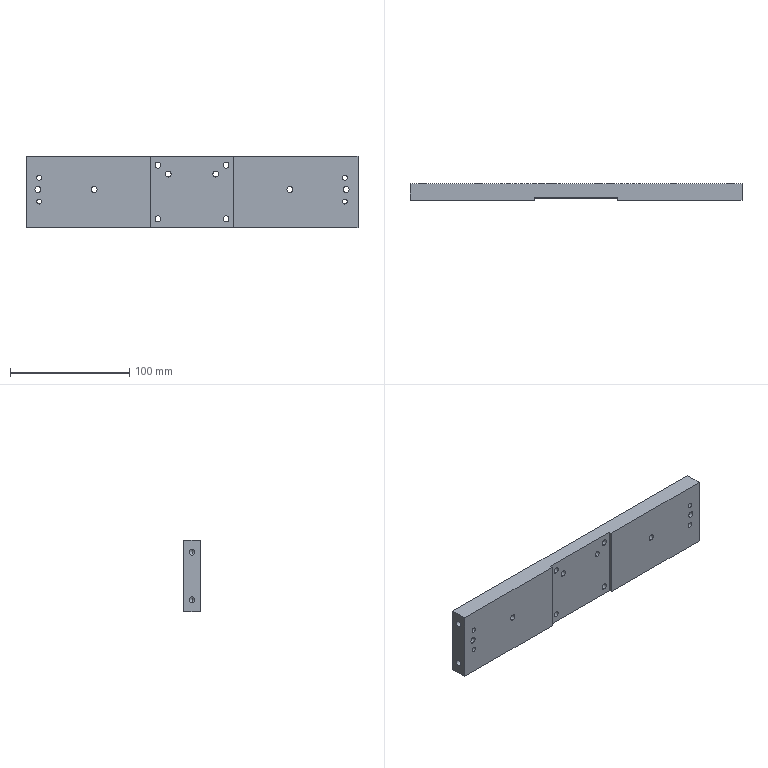Component | SolidWorks | OPW-05-003-1 | 1 solid | 54 faces | box 278 x 14 x 60 mm | volume 220456 mm3 | cylinder 36 | plane 10 | cone 8 | commonest cylinder face diameters 5 x28 4.2 x8
build123d program:
from build123d import *

# Parameters (mm, degrees)
SKETCH1_W                  = 278
SKETCH1_H                  = 60
BOSS_EXTRUDE1_DEPTH        = 7
M6_TAPPED_HOLE1_AT_2_COUNT = 2
M6_TAPPED_HOLE1_AT_2_PITCH = 40
SKETCH6_W                  = 70
SKETCH6_H                  = 60
CUT_EXTRUDE1_DEPTH         = 2
M5_TAPPED_HOLE1_D          = 4.2
M5_TAPPED_HOLE1_DEPTH      = 14
M5_TAPPED_HOLE1_TIP        = 1.262
M6_TAPPED_HOLE2_D          = 5
M6_TAPPED_HOLE2_DEPTH      = 17
M6_TAPPED_HOLE2_TIP        = 1.502
M6_TAPPED_HOLE5_D          = 5
M6_TAPPED_HOLE5_DEPTH      = 15
M6_TAPPED_HOLE5_TIP        = 1.502
M6_TAPPED_HOLE6_D          = 5


with BuildPart() as part:
    # Sketch1 → Boss-Extrude1 (new, symmetric)
    with BuildSketch(Plane(origin=(0, 0, 0), x_dir=(1, 0, 0), z_dir=(0, 1, 0))):
        Rectangle(SKETCH1_W, SKETCH1_H)
    extrude(amount=BOSS_EXTRUDE1_DEPTH, both=True)

    # Sketch4 → M6 Tapped Hole1 (revolve, cut)
    with BuildSketch(Plane(origin=(-139, 0, -20), x_dir=(0, 0, 1), z_dir=(0, 1, 0))):
        Polygon((0, 0), (0, 18.502), (2.5, 17), (2.5, 0), align=None)
    m6_tapped_hole1 = revolve(axis=Axis((-145.35, 0, -20), (1, 0, 0)), mode=Mode.SUBTRACT)

    # M6 Tapped Hole1 at 2: M6 Tapped Hole1 ×2
    with Locations(*[(0, 0, i * M6_TAPPED_HOLE1_AT_2_PITCH) for i in range(1, M6_TAPPED_HOLE1_AT_2_COUNT)]):
        add(m6_tapped_hole1, mode=Mode.SUBTRACT)

    # Mirror1: M6 Tapped Hole1 across plane
    add(m6_tapped_hole1.mirror(Plane(origin=(0, 0, 0), x_dir=(0, 0, 1), z_dir=(1, 0, 0))), mode=Mode.SUBTRACT)

    # Mirror1 copy 1 sketch → Mirror1 copy 1 (revolve, cut)
    with BuildSketch(Plane(origin=(139, 0, 20), x_dir=(0, 0, 1), z_dir=(0, 1, 0))):
        Polygon((0, 0), (0, -18.502), (2.5, -17), (2.5, 0), align=None)
    revolve(axis=Axis((145.35, 0, 20), (1, 0, 0)), mode=Mode.SUBTRACT)

    # Sketch6 → Cut-Extrude1 (cut)
    with BuildSketch(Plane.XZ.offset(7)):
        Rectangle(SKETCH6_W, SKETCH6_H)
    extrude(amount=-CUT_EXTRUDE1_DEPTH, mode=Mode.SUBTRACT)

    # M5 Tapped Hole1
    with Locations(Plane(origin=(0, 7, 0), x_dir=(-1, 0, 0), z_dir=(0, 1, 0))):
        with Locations((128, 12), (128, -8), (-128, -8), (-128, 12)):
            Hole(M5_TAPPED_HOLE1_D / 2, depth=M5_TAPPED_HOLE1_DEPTH)
            with Locations((0, 0, -(M5_TAPPED_HOLE1_DEPTH + M5_TAPPED_HOLE1_TIP / 2))):  # 118° drill point
                Cone(0, M5_TAPPED_HOLE1_D / 2, M5_TAPPED_HOLE1_TIP, mode=Mode.SUBTRACT)

    # M6 Tapped Hole2
    with Locations(Plane(origin=(0, 7, 0), x_dir=(-1, 0, 0), z_dir=(0, 1, 0))):
        with Locations((20, 15), (-20, 15)):
            Hole(M6_TAPPED_HOLE2_D / 2, depth=M6_TAPPED_HOLE2_DEPTH)
            with Locations((0, 0, -(M6_TAPPED_HOLE2_DEPTH + M6_TAPPED_HOLE2_TIP / 2))):  # 118° drill point
                Cone(0, M6_TAPPED_HOLE2_D / 2, M6_TAPPED_HOLE2_TIP, mode=Mode.SUBTRACT)

    # M6 Tapped Hole5
    with Locations(Plane.XZ.offset(5)):
        with Locations((28.5, -22.5), (-28.5, -22.5), (-28.5, 22.5), (28.5, 22.5)):
            Hole(M6_TAPPED_HOLE5_D / 2, depth=M6_TAPPED_HOLE5_DEPTH)
            with Locations((0, 0, -(M6_TAPPED_HOLE5_DEPTH + M6_TAPPED_HOLE5_TIP / 2))):  # 118° drill point
                Cone(0, M6_TAPPED_HOLE5_D / 2, M6_TAPPED_HOLE5_TIP, mode=Mode.SUBTRACT)

    # M6 Tapped Hole6 (through all)
    with Locations(Plane.XZ.offset(7)):
        with Locations((129, 2), (82, 2)):
            m6_tapped_hole6 = Hole(M6_TAPPED_HOLE6_D / 2)

    # Mirror3: M6 Tapped Hole6 across plane
    add(m6_tapped_hole6.mirror(Plane(origin=(0, 0, 0), x_dir=(0, 0, 1), z_dir=(1, 0, 0))), mode=Mode.SUBTRACT)


solid = part.part

# Placed as in the assembly
solid = solid.moved(Location((-104.904, 48.999, 0), (0, 0, 0)))